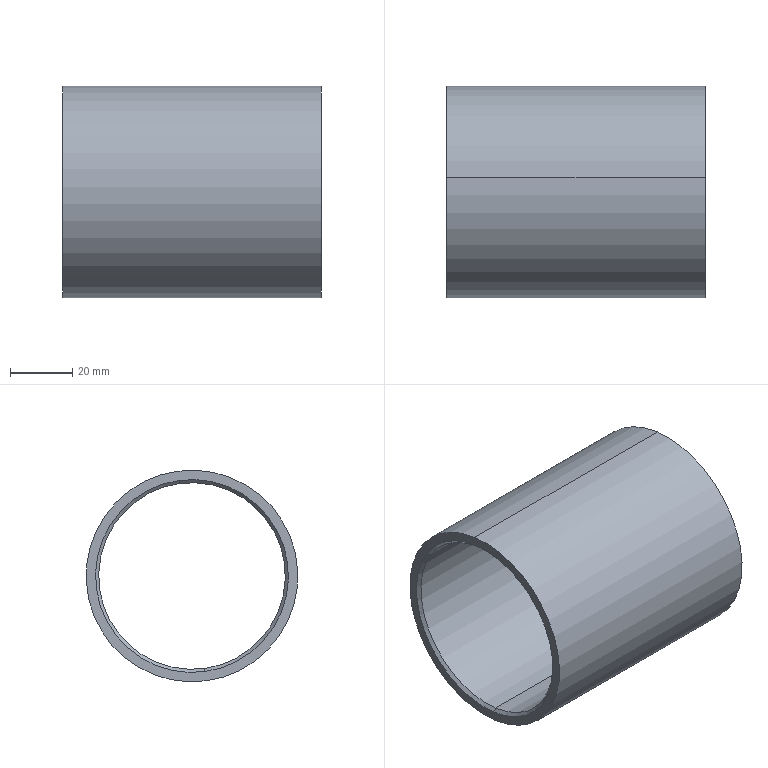Component | SolidWorks | SpindleSleeve1-1 | 1 solid | 10 faces | box 83 x 68 x 68 mm | volume 66562 mm3 | cone 4 | cylinder 4 | plane 2 | commonest cylinder face diameters 60 x2 68 x2
build123d program:
from build123d import *

# Parameters (mm, degrees)
SKETCH1_R           = 34
SKETCH1_R_2         = 30
BOSS_EXTRUDE1_DEPTH = 41.5
CHAMFER1_SIZE       = 1


with BuildPart() as part:
    # Sketch1 → Boss-Extrude1 (new, symmetric)
    with BuildSketch(Plane(origin=(0, 0, 0), x_dir=(0, 0, -1), z_dir=(1, 0, 0))):
        Circle(SKETCH1_R)
        Circle(SKETCH1_R_2, mode=Mode.SUBTRACT)
    extrude(amount=BOSS_EXTRUDE1_DEPTH, both=True)

    # Chamfer1
    chamfer1_edges = [part.edges().sort_by_distance(p)[0] for p in [
        (-41.5, 0, 30),
        (41.5, 0, 30),
    ]]
    chamfer(chamfer1_edges, length=CHAMFER1_SIZE)


solid = part.part

# Placed as in the assembly
solid = solid.moved(Location((622.803, 34.532, 0), (0, 0, 0)))
STEP:
#1=CARTESIAN_POINT('',(26.114,1.516,1.171));
#2=VERTEX_POINT('',#1);
#3=CARTESIAN_POINT('',(26.114,1.203,-1.171));
#4=VERTEX_POINT('',#3);
#5=CARTESIAN_POINT('',(26.114,1.36,0.));
#6=DIRECTION('',(1.,0.,0.));
#7=DIRECTION('',(0.,-0.1329,-0.9911));
#8=AXIS2_PLACEMENT_3D('',#5,#6,#7);
#9=CIRCLE('',#8,1.181);
#10=EDGE_CURVE('',#2,#4,#9,.T.);
#11=ORIENTED_EDGE('',*,*,#10,.F.);
#12=CARTESIAN_POINT('',(26.154,1.522,1.21));
#13=VERTEX_POINT('',#12);
#14=CARTESIAN_POINT('',(26.114,1.516,1.171));
#15=DIRECTION('',(0.7071,0.09394,0.7008));
#16=VECTOR('',#15,39.37);
#17=LINE('',#14,#16);
#18=EDGE_CURVE('',#2,#13,#17,.T.);
#19=ORIENTED_EDGE('',*,*,#18,.T.);
#20=CARTESIAN_POINT('',(26.154,1.197,-1.21));
#21=VERTEX_POINT('',#20);
#22=CARTESIAN_POINT('',(26.154,1.36,0.));
#23=DIRECTION('',(-1.,0.,0.));
#24=DIRECTION('',(0.,-0.1329,-0.9911));
#25=AXIS2_PLACEMENT_3D('',#22,#23,#24);
#26=CIRCLE('',#25,1.22);
#27=EDGE_CURVE('',#21,#13,#26,.T.);
#28=ORIENTED_EDGE('',*,*,#27,.F.);
#29=CARTESIAN_POINT('',(26.114,1.203,-1.171));
#30=DIRECTION('',(0.7071,-0.09394,-0.7008));
#31=VECTOR('',#30,39.37);
#32=LINE('',#29,#31);
#33=EDGE_CURVE('',#4,#21,#32,.T.);
#34=ORIENTED_EDGE('',*,*,#33,.F.);
#35=EDGE_LOOP('',(#11,#19,#28,#34));
#36=FACE_OUTER_BOUND('',#35,.T.);
#37=CARTESIAN_POINT('',(26.114,1.36,0.));
#38=DIRECTION('',(1.,0.,0.));
#39=DIRECTION('',(0.,-0.1329,-0.9911));
#40=AXIS2_PLACEMENT_3D('',#37,#38,#39);
#41=CONICAL_SURFACE('',#40,1.181,0.7854);
#42=ADVANCED_FACE('',(#36),#41,.F.);
#43=CARTESIAN_POINT('',(22.925,1.203,-1.171));
#44=VERTEX_POINT('',#43);
#45=CARTESIAN_POINT('',(22.925,1.516,1.171));
#46=VERTEX_POINT('',#45);
#47=CARTESIAN_POINT('',(22.925,1.36,0.));
#48=DIRECTION('',(-1.,0.,0.));
#49=DIRECTION('',(0.,-0.1329,-0.9911));
#50=AXIS2_PLACEMENT_3D('',#47,#48,#49);
#51=CIRCLE('',#50,1.181);
#52=EDGE_CURVE('',#44,#46,#51,.T.);
#53=ORIENTED_EDGE('',*,*,#52,.F.);
#54=CARTESIAN_POINT('',(22.886,1.197,-1.21));
#55=VERTEX_POINT('',#54);
#56=CARTESIAN_POINT('',(22.886,1.197,-1.21));
#57=DIRECTION('',(-0.7071,-0.09394,-0.7008));
#58=VECTOR('',#57,39.37);
#59=LINE('',#56,#58);
#60=EDGE_CURVE('',#44,#55,#59,.T.);
#61=ORIENTED_EDGE('',*,*,#60,.T.);
#62=CARTESIAN_POINT('',(22.886,1.522,1.21));
#63=VERTEX_POINT('',#62);
#64=CARTESIAN_POINT('',(22.886,1.36,0.));
#65=DIRECTION('',(1.,0.,0.));
#66=DIRECTION('',(0.,-0.1329,-0.9911));
#67=AXIS2_PLACEMENT_3D('',#64,#65,#66);
#68=CIRCLE('',#67,1.22);
#69=EDGE_CURVE('',#63,#55,#68,.T.);
#70=ORIENTED_EDGE('',*,*,#69,.F.);
#71=CARTESIAN_POINT('',(22.886,1.522,1.21));
#72=DIRECTION('',(-0.7071,0.09394,0.7008));
#73=VECTOR('',#72,39.37);
#74=LINE('',#71,#73);
#75=EDGE_CURVE('',#46,#63,#74,.T.);
#76=ORIENTED_EDGE('',*,*,#75,.F.);
#77=EDGE_LOOP('',(#53,#61,#70,#76));
#78=FACE_OUTER_BOUND('',#77,.T.);
#79=CARTESIAN_POINT('',(22.886,1.36,0.));
#80=DIRECTION('',(-1.,0.,0.));
#81=DIRECTION('',(0.,0.1329,0.9911));
#82=AXIS2_PLACEMENT_3D('',#79,#80,#81);
#83=CONICAL_SURFACE('',#82,1.22,0.7854);
#84=ADVANCED_FACE('',(#78),#83,.F.);
#85=ORIENTED_EDGE('',*,*,#10,.T.);
#86=CARTESIAN_POINT('',(26.154,1.203,-1.171));
#87=DIRECTION('',(-1.,0.,0.));
#88=VECTOR('',#87,39.37);
#89=LINE('',#86,#88);
#90=EDGE_CURVE('',#4,#44,#89,.T.);
#91=ORIENTED_EDGE('',*,*,#90,.T.);
#92=ORIENTED_EDGE('',*,*,#52,.T.);
#93=CARTESIAN_POINT('',(26.154,1.516,1.171));
#94=DIRECTION('',(-1.,0.,0.));
#95=VECTOR('',#94,39.37);
#96=LINE('',#93,#95);
#97=EDGE_CURVE('',#2,#46,#96,.T.);
#98=ORIENTED_EDGE('',*,*,#97,.F.);
#99=EDGE_LOOP('',(#85,#91,#92,#98));
#100=FACE_OUTER_BOUND('',#99,.T.);
#101=CARTESIAN_POINT('',(26.154,1.36,0.));
#102=DIRECTION('',(-1.,0.,0.));
#103=DIRECTION('',(0.,0.1329,0.9911));
#104=AXIS2_PLACEMENT_3D('',#101,#102,#103);
#105=CYLINDRICAL_SURFACE('',#104,1.181);
#106=ADVANCED_FACE('',(#100),#105,.F.);
#107=CARTESIAN_POINT('',(26.154,1.182,-1.327));
#108=VERTEX_POINT('',#107);
#109=CARTESIAN_POINT('',(26.154,1.537,1.327));
#110=VERTEX_POINT('',#109);
#111=CARTESIAN_POINT('',(26.154,1.36,0.));
#112=DIRECTION('',(1.,0.,0.));
#113=DIRECTION('',(0.,-0.1329,-0.9911));
#114=AXIS2_PLACEMENT_3D('',#111,#112,#113);
#115=CIRCLE('',#114,1.339);
#116=EDGE_CURVE('',#108,#110,#115,.T.);
#117=ORIENTED_EDGE('',*,*,#116,.F.);
#118=CARTESIAN_POINT('',(22.886,1.182,-1.327));
#119=VERTEX_POINT('',#118);
#120=CARTESIAN_POINT('',(26.154,1.182,-1.327));
#121=DIRECTION('',(-1.,0.,0.));
#122=VECTOR('',#121,39.37);
#123=LINE('',#120,#122);
#124=EDGE_CURVE('',#108,#119,#123,.T.);
#125=ORIENTED_EDGE('',*,*,#124,.T.);
#126=CARTESIAN_POINT('',(22.886,1.537,1.327));
#127=VERTEX_POINT('',#126);
#128=CARTESIAN_POINT('',(22.886,1.36,0.));
#129=DIRECTION('',(1.,0.,0.));
#130=DIRECTION('',(0.,-0.1329,-0.9911));
#131=AXIS2_PLACEMENT_3D('',#128,#129,#130);
#132=CIRCLE('',#131,1.339);
#133=EDGE_CURVE('',#119,#127,#132,.T.);
#134=ORIENTED_EDGE('',*,*,#133,.T.);
#135=CARTESIAN_POINT('',(26.154,1.537,1.327));
#136=DIRECTION('',(-1.,0.,0.));
#137=VECTOR('',#136,39.37);
#138=LINE('',#135,#137);
#139=EDGE_CURVE('',#110,#127,#138,.T.);
#140=ORIENTED_EDGE('',*,*,#139,.F.);
#141=EDGE_LOOP('',(#117,#125,#134,#140));
#142=FACE_OUTER_BOUND('',#141,.T.);
#143=CARTESIAN_POINT('',(26.154,1.36,0.));
#144=DIRECTION('',(-1.,0.,0.));
#145=DIRECTION('',(0.,0.1329,0.9911));
#146=AXIS2_PLACEMENT_3D('',#143,#144,#145);
#147=CYLINDRICAL_SURFACE('',#146,1.339);
#148=ADVANCED_FACE('',(#142),#147,.T.);
#149=ORIENTED_EDGE('',*,*,#27,.T.);
#150=CARTESIAN_POINT('',(26.154,1.36,0.));
#151=DIRECTION('',(-1.,0.,0.));
#152=DIRECTION('',(0.,-0.1329,-0.9911));
#153=AXIS2_PLACEMENT_3D('',#150,#151,#152);
#154=CIRCLE('',#153,1.22);
#155=EDGE_CURVE('',#13,#21,#154,.T.);
#156=ORIENTED_EDGE('',*,*,#155,.T.);
#157=EDGE_LOOP('',(#149,#156));
#158=FACE_BOUND('',#157,.T.);
#159=CARTESIAN_POINT('',(26.154,1.36,0.));
#160=DIRECTION('',(1.,0.,0.));
#161=DIRECTION('',(0.,-0.1329,-0.9911));
#162=AXIS2_PLACEMENT_3D('',#159,#160,#161);
#163=CIRCLE('',#162,1.339);
#164=EDGE_CURVE('',#110,#108,#163,.T.);
#165=ORIENTED_EDGE('',*,*,#164,.T.);
#166=ORIENTED_EDGE('',*,*,#116,.T.);
#167=EDGE_LOOP('',(#165,#166));
#168=FACE_OUTER_BOUND('',#167,.T.);
#169=CARTESIAN_POINT('',(26.154,1.36,0.));
#170=DIRECTION('',(1.,0.,0.));
#171=DIRECTION('',(0.,-0.1329,-0.9911));
#172=AXIS2_PLACEMENT_3D('',#169,#170,#171);
#173=PLANE('',#172);
#174=ADVANCED_FACE('',(#158,#168),#173,.T.);
#175=ORIENTED_EDGE('',*,*,#69,.T.);
#176=CARTESIAN_POINT('',(22.886,1.36,0.));
#177=DIRECTION('',(1.,0.,0.));
#178=DIRECTION('',(0.,-0.1329,-0.9911));
#179=AXIS2_PLACEMENT_3D('',#176,#177,#178);
#180=CIRCLE('',#179,1.22);
#181=EDGE_CURVE('',#55,#63,#180,.T.);
#182=ORIENTED_EDGE('',*,*,#181,.T.);
#183=EDGE_LOOP('',(#175,#182));
#184=FACE_BOUND('',#183,.T.);
#185=CARTESIAN_POINT('',(22.886,1.36,0.));
#186=DIRECTION('',(1.,0.,0.));
#187=DIRECTION('',(0.,-0.1329,-0.9911));
#188=AXIS2_PLACEMENT_3D('',#185,#186,#187);
#189=CIRCLE('',#188,1.339);
#190=EDGE_CURVE('',#127,#119,#189,.T.);
#191=ORIENTED_EDGE('',*,*,#190,.F.);
#192=ORIENTED_EDGE('',*,*,#133,.F.);
#193=EDGE_LOOP('',(#191,#192));
#194=FACE_OUTER_BOUND('',#193,.T.);
#195=CARTESIAN_POINT('',(22.886,1.36,0.));
#196=DIRECTION('',(1.,0.,0.));
#197=DIRECTION('',(0.,-0.1329,-0.9911));
#198=AXIS2_PLACEMENT_3D('',#195,#196,#197);
#199=PLANE('',#198);
#200=ADVANCED_FACE('',(#184,#194),#199,.F.);
#201=ORIENTED_EDGE('',*,*,#124,.F.);
#202=ORIENTED_EDGE('',*,*,#164,.F.);
#203=ORIENTED_EDGE('',*,*,#139,.T.);
#204=ORIENTED_EDGE('',*,*,#190,.T.);
#205=EDGE_LOOP('',(#201,#202,#203,#204));
#206=FACE_OUTER_BOUND('',#205,.T.);
#207=CARTESIAN_POINT('',(26.154,1.36,0.));
#208=DIRECTION('',(-1.,0.,0.));
#209=DIRECTION('',(0.,0.1329,0.9911));
#210=AXIS2_PLACEMENT_3D('',#207,#208,#209);
#211=CYLINDRICAL_SURFACE('',#210,1.339);
#212=ADVANCED_FACE('',(#206),#211,.T.);
#213=ORIENTED_EDGE('',*,*,#90,.F.);
#214=CARTESIAN_POINT('',(26.114,1.36,0.));
#215=DIRECTION('',(1.,0.,0.));
#216=DIRECTION('',(0.,-0.1329,-0.9911));
#217=AXIS2_PLACEMENT_3D('',#214,#215,#216);
#218=CIRCLE('',#217,1.181);
#219=EDGE_CURVE('',#4,#2,#218,.T.);
#220=ORIENTED_EDGE('',*,*,#219,.T.);
#221=ORIENTED_EDGE('',*,*,#97,.T.);
#222=CARTESIAN_POINT('',(22.925,1.36,0.));
#223=DIRECTION('',(-1.,0.,0.));
#224=DIRECTION('',(0.,-0.1329,-0.9911));
#225=AXIS2_PLACEMENT_3D('',#222,#223,#224);
#226=CIRCLE('',#225,1.181);
#227=EDGE_CURVE('',#46,#44,#226,.T.);
#228=ORIENTED_EDGE('',*,*,#227,.T.);
#229=EDGE_LOOP('',(#213,#220,#221,#228));
#230=FACE_OUTER_BOUND('',#229,.T.);
#231=CARTESIAN_POINT('',(26.154,1.36,0.));
#232=DIRECTION('',(-1.,0.,0.));
#233=DIRECTION('',(0.,0.1329,0.9911));
#234=AXIS2_PLACEMENT_3D('',#231,#232,#233);
#235=CYLINDRICAL_SURFACE('',#234,1.181);
#236=ADVANCED_FACE('',(#230),#235,.F.);
#237=ORIENTED_EDGE('',*,*,#60,.F.);
#238=ORIENTED_EDGE('',*,*,#227,.F.);
#239=ORIENTED_EDGE('',*,*,#75,.T.);
#240=ORIENTED_EDGE('',*,*,#181,.F.);
#241=EDGE_LOOP('',(#237,#238,#239,#240));
#242=FACE_OUTER_BOUND('',#241,.T.);
#243=CARTESIAN_POINT('',(22.886,1.36,0.));
#244=DIRECTION('',(-1.,0.,0.));
#245=DIRECTION('',(0.,0.1329,0.9911));
#246=AXIS2_PLACEMENT_3D('',#243,#244,#245);
#247=CONICAL_SURFACE('',#246,1.22,0.7854);
#248=ADVANCED_FACE('',(#242),#247,.F.);
#249=ORIENTED_EDGE('',*,*,#18,.F.);
#250=ORIENTED_EDGE('',*,*,#219,.F.);
#251=ORIENTED_EDGE('',*,*,#33,.T.);
#252=ORIENTED_EDGE('',*,*,#155,.F.);
#253=EDGE_LOOP('',(#249,#250,#251,#252));
#254=FACE_OUTER_BOUND('',#253,.T.);
#255=CARTESIAN_POINT('',(26.114,1.36,0.));
#256=DIRECTION('',(1.,0.,0.));
#257=DIRECTION('',(0.,-0.1329,-0.9911));
#258=AXIS2_PLACEMENT_3D('',#255,#256,#257);
#259=CONICAL_SURFACE('',#258,1.181,0.7854);
#260=ADVANCED_FACE('',(#254),#259,.F.);
#261=CLOSED_SHELL('',(#42,#84,#106,#148,#174,#200,#212,#236,#248,#260));
#262=MANIFOLD_SOLID_BREP('',#261);
#263=CARTESIAN_POINT('',(0.,0.,0.));
#264=DIRECTION('',(0.,0.,1.));
#265=DIRECTION('',(1.,0.,0.));
#266=AXIS2_PLACEMENT_3D('',#263,#264,#265);
#267=(LENGTH_UNIT()NAMED_UNIT(*)SI_UNIT($,.METRE.));
#268=LENGTH_MEASURE_WITH_UNIT(LENGTH_MEASURE(0.0254),#267);
#269=DIMENSIONAL_EXPONENTS(1.,0.,0.,0.,0.,0.,0.);
#270=(CONVERSION_BASED_UNIT('',#268)LENGTH_UNIT()NAMED_UNIT(#269));
#271=UNCERTAINTY_MEASURE_WITH_UNIT(LENGTH_MEASURE(0.00001),#270,'','');
#272=(NAMED_UNIT(*)PLANE_ANGLE_UNIT()SI_UNIT($,.RADIAN.));
#273=(NAMED_UNIT(*)SI_UNIT($,.STERADIAN.)SOLID_ANGLE_UNIT());
#274=(GEOMETRIC_REPRESENTATION_CONTEXT(3)GLOBAL_UNCERTAINTY_ASSIGNED_CONTEXT((#271))GLOBAL_UNIT_ASSIGNED_CONTEXT((#270,#272,#273))REPRESENTATION_CONTEXT('',''));
#275=ADVANCED_BREP_SHAPE_REPRESENTATION('',(#262,#266),#274);
#276=COLOUR_RGB('',0.7922,0.8196,0.9333);
#277=FILL_AREA_STYLE_COLOUR('',#276);
#278=FILL_AREA_STYLE('',(#277));
#279=SURFACE_STYLE_FILL_AREA(#278);
#280=SURFACE_SIDE_STYLE('',(#279));
#281=SURFACE_STYLE_USAGE(.BOTH.,#280);
#282=PRESENTATION_STYLE_ASSIGNMENT((#281));
#283=STYLED_ITEM('',(#282),#262);
#284=PRESENTATION_LAYER_ASSIGNMENT('','',(#283));
#285=(LENGTH_UNIT()NAMED_UNIT(*)SI_UNIT($,.METRE.));
#286=LENGTH_MEASURE_WITH_UNIT(LENGTH_MEASURE(0.0254),#285);
#287=DIMENSIONAL_EXPONENTS(1.,0.,0.,0.,0.,0.,0.);
#288=(CONVERSION_BASED_UNIT('',#286)LENGTH_UNIT()NAMED_UNIT(#287));
#289=UNCERTAINTY_MEASURE_WITH_UNIT(LENGTH_MEASURE(0.00001),#288,'','');
#290=(NAMED_UNIT(*)PLANE_ANGLE_UNIT()SI_UNIT($,.RADIAN.));
#291=(NAMED_UNIT(*)SI_UNIT($,.STERADIAN.)SOLID_ANGLE_UNIT());
#292=(GEOMETRIC_REPRESENTATION_CONTEXT(3)GLOBAL_UNCERTAINTY_ASSIGNED_CONTEXT((#289))GLOBAL_UNIT_ASSIGNED_CONTEXT((#288,#290,#291))REPRESENTATION_CONTEXT('',''));
#293=MECHANICAL_DESIGN_GEOMETRIC_PRESENTATION_REPRESENTATION('',(#283),#292);